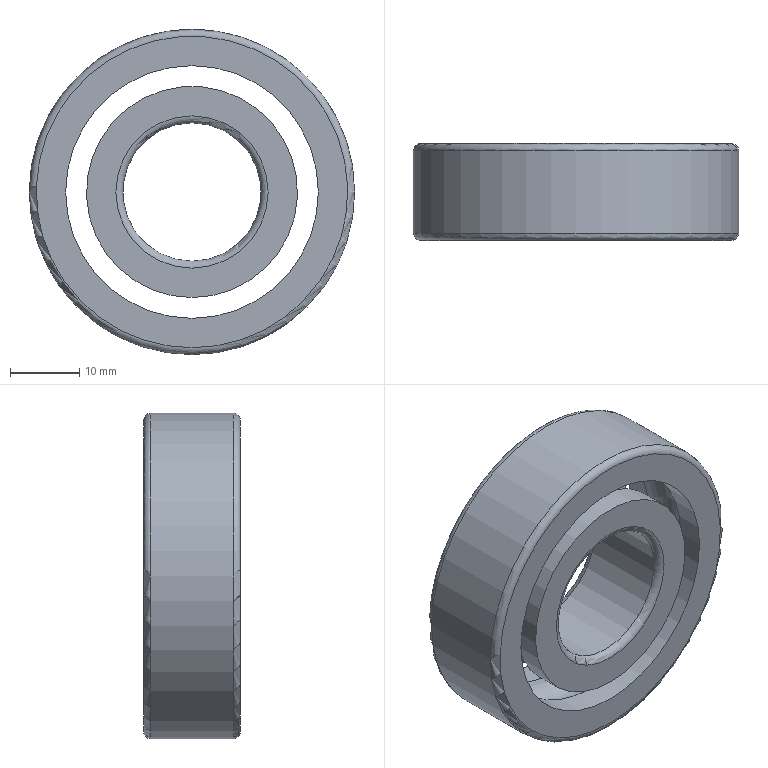Component | NX | GUNDONGZHOUCHENG9 | 2 solids | 16 faces | box 47 x 14 x 47 mm | volume 13471 mm3 | torus 6 | cylinder 6 | plane 4 | commonest cylinder face diameters 36.5 x2 30.5 x2 47 x1 20 x1
STEP:
#1=CARTESIAN_POINT('',(0.,0.,0.));
#2=DIRECTION('',(0.,0.,1.));
#3=DIRECTION('',(1.,0.,0.));
#4=AXIS2_PLACEMENT_3D('',#1,#2,#3);
#5=CARTESIAN_POINT('',(0.,0.,-22.5));
#6=VERTEX_POINT('',#5);
#7=CARTESIAN_POINT('',(0.,0.,0.));
#8=DIRECTION('',(0.,-1.,0.));
#9=DIRECTION('',(0.,0.,-1.));
#10=AXIS2_PLACEMENT_3D('',#7,#8,#9);
#11=CIRCLE('',#10,22.5);
#12=CARTESIAN_POINT('',(0.,1.,0.));
#13=DIRECTION('',(0.,-1.,0.));
#14=DIRECTION('',(0.,0.,-1.));
#15=AXIS2_PLACEMENT_3D('',#12,#13,#14);
#16=TOROIDAL_SURFACE('',#15,22.5,1.);
#17=CARTESIAN_POINT('',(0.,7.854));
#18=DIRECTION('',(1.,0.));
#19=VECTOR('',#18,1.);
#20=LINE('',#17,#19);
#21=(GEOMETRIC_REPRESENTATION_CONTEXT(2)PARAMETRIC_REPRESENTATION_CONTEXT()REPRESENTATION_CONTEXT('',''));
#22=DEFINITIONAL_REPRESENTATION('',(#20),#21);
#23=PCURVE('',#16,#22);
#24=CARTESIAN_POINT('',(22.5,0.,0.));
#25=DIRECTION('',(0.,1.,0.));
#26=DIRECTION('',(0.,0.,1.));
#27=AXIS2_PLACEMENT_3D('',#24,#25,#26);
#28=PLANE('',#27);
#29=CARTESIAN_POINT('',(-22.5,-22.5));
#30=CARTESIAN_POINT('',(-22.5,16.471));
#31=CARTESIAN_POINT('',(11.25,-3.014));
#32=CARTESIAN_POINT('',(45.,-22.5));
#33=CARTESIAN_POINT('',(11.25,-41.986));
#34=CARTESIAN_POINT('',(-22.5,-61.471));
#35=CARTESIAN_POINT('',(-22.5,-22.5));
#36=(BOUNDED_CURVE()B_SPLINE_CURVE(2,(#29,#30,#31,#32,#33,#34,#35),.UNSPECIFIED.,.T.,.F.)B_SPLINE_CURVE_WITH_KNOTS((1,2,2,2,2,1),(-2.094,0.,2.094,4.189,6.283,8.378),.UNSPECIFIED.)CURVE()GEOMETRIC_REPRESENTATION_ITEM()RATIONAL_B_SPLINE_CURVE((1.,0.5,1.,0.5,1.,0.5,1.))REPRESENTATION_ITEM(''));
#37=(GEOMETRIC_REPRESENTATION_CONTEXT(2)PARAMETRIC_REPRESENTATION_CONTEXT()REPRESENTATION_CONTEXT('',''));
#38=DEFINITIONAL_REPRESENTATION('',(#36),#37);
#39=PCURVE('',#28,#38);
#40=SURFACE_CURVE('',#11,(#23,#39),.PCURVE_S1.);
#41=EDGE_CURVE('',#6,#6,#40,.T.);
#42=ORIENTED_EDGE('',*,*,#41,.F.);
#43=CARTESIAN_POINT('',(0.,1.,-23.5));
#44=VERTEX_POINT('',#43);
#45=CARTESIAN_POINT('',(-0.,1.,-23.5));
#46=CARTESIAN_POINT('',(-0.,0.7327,-23.5));
#47=CARTESIAN_POINT('',(-0.,0.4723,-23.415));
#48=CARTESIAN_POINT('',(-0.,0.2481,-23.252));
#49=CARTESIAN_POINT('',(-0.,0.085,-23.028));
#50=CARTESIAN_POINT('',(-0.,0.,-22.767));
#51=CARTESIAN_POINT('',(-0.,0.,-22.5));
#52=(BOUNDED_CURVE()B_SPLINE_CURVE(6,(#45,#46,#47,#48,#49,#50,#51),.UNSPECIFIED.,.F.,.F.)B_SPLINE_CURVE_WITH_KNOTS((7,7),(0.,1.571),.PIECEWISE_BEZIER_KNOTS.)CURVE()GEOMETRIC_REPRESENTATION_ITEM()RATIONAL_B_SPLINE_CURVE((1.031,1.01,0.9979,0.994,0.9979,1.01,1.031))REPRESENTATION_ITEM(''));
#53=CARTESIAN_POINT('',(0.,6.283));
#54=DIRECTION('',(0.,1.));
#55=VECTOR('',#54,1.);
#56=LINE('',#53,#55);
#57=(GEOMETRIC_REPRESENTATION_CONTEXT(2)PARAMETRIC_REPRESENTATION_CONTEXT()REPRESENTATION_CONTEXT('',''));
#58=DEFINITIONAL_REPRESENTATION('',(#56),#57);
#59=PCURVE('',#16,#58);
#60=CARTESIAN_POINT('',(6.283,6.283));
#61=DIRECTION('',(0.,1.));
#62=VECTOR('',#61,1.);
#63=LINE('',#60,#62);
#64=(GEOMETRIC_REPRESENTATION_CONTEXT(2)PARAMETRIC_REPRESENTATION_CONTEXT()REPRESENTATION_CONTEXT('',''));
#65=DEFINITIONAL_REPRESENTATION('',(#63),#64);
#66=PCURVE('',#16,#65);
#67=SEAM_CURVE('',#52,(#59,#66),.PCURVE_S1.);
#68=EDGE_CURVE('',#44,#6,#67,.T.);
#69=ORIENTED_EDGE('',*,*,#68,.F.);
#70=CARTESIAN_POINT('',(0.,1.,0.));
#71=DIRECTION('',(0.,-1.,0.));
#72=DIRECTION('',(0.,0.,-1.));
#73=AXIS2_PLACEMENT_3D('',#70,#71,#72);
#74=CIRCLE('',#73,23.5);
#75=CARTESIAN_POINT('',(0.,6.283));
#76=DIRECTION('',(1.,0.));
#77=VECTOR('',#76,1.);
#78=LINE('',#75,#77);
#79=(GEOMETRIC_REPRESENTATION_CONTEXT(2)PARAMETRIC_REPRESENTATION_CONTEXT()REPRESENTATION_CONTEXT('',''));
#80=DEFINITIONAL_REPRESENTATION('',(#78),#79);
#81=PCURVE('',#16,#80);
#82=CARTESIAN_POINT('',(0.,0.,0.));
#83=DIRECTION('',(0.,-1.,0.));
#84=DIRECTION('',(0.,0.,-1.));
#85=AXIS2_PLACEMENT_3D('',#82,#83,#84);
#86=CYLINDRICAL_SURFACE('',#85,23.5);
#87=CARTESIAN_POINT('',(0.,-1.));
#88=DIRECTION('',(1.,0.));
#89=VECTOR('',#88,1.);
#90=LINE('',#87,#89);
#91=(GEOMETRIC_REPRESENTATION_CONTEXT(2)PARAMETRIC_REPRESENTATION_CONTEXT()REPRESENTATION_CONTEXT('',''));
#92=DEFINITIONAL_REPRESENTATION('',(#90),#91);
#93=PCURVE('',#86,#92);
#94=SURFACE_CURVE('',#74,(#81,#93),.PCURVE_S1.);
#95=EDGE_CURVE('',#44,#44,#94,.T.);
#96=ORIENTED_EDGE('',*,*,#95,.T.);
#97=ORIENTED_EDGE('',*,*,#68,.T.);
#98=EDGE_LOOP('',(#42,#69,#96,#97));
#99=FACE_BOUND('',#98,.T.);
#100=ADVANCED_FACE('',(#99),#16,.T.);
#101=CARTESIAN_POINT('',(0.,0.,-18.25));
#102=VERTEX_POINT('',#101);
#103=CARTESIAN_POINT('',(0.,0.,0.));
#104=DIRECTION('',(0.,-1.,0.));
#105=DIRECTION('',(0.,0.,-1.));
#106=AXIS2_PLACEMENT_3D('',#103,#104,#105);
#107=CIRCLE('',#106,18.25);
#108=CARTESIAN_POINT('',(-18.25,-22.5));
#109=CARTESIAN_POINT('',(-18.25,9.11));
#110=CARTESIAN_POINT('',(9.125,-6.695));
#111=CARTESIAN_POINT('',(36.5,-22.5));
#112=CARTESIAN_POINT('',(9.125,-38.305));
#113=CARTESIAN_POINT('',(-18.25,-54.11));
#114=CARTESIAN_POINT('',(-18.25,-22.5));
#115=(BOUNDED_CURVE()B_SPLINE_CURVE(2,(#108,#109,#110,#111,#112,#113,#114),.UNSPECIFIED.,.T.,.F.)B_SPLINE_CURVE_WITH_KNOTS((1,2,2,2,2,1),(-2.094,0.,2.094,4.189,6.283,8.378),.UNSPECIFIED.)CURVE()GEOMETRIC_REPRESENTATION_ITEM()RATIONAL_B_SPLINE_CURVE((1.,0.5,1.,0.5,1.,0.5,1.))REPRESENTATION_ITEM(''));
#116=(GEOMETRIC_REPRESENTATION_CONTEXT(2)PARAMETRIC_REPRESENTATION_CONTEXT()REPRESENTATION_CONTEXT('',''));
#117=DEFINITIONAL_REPRESENTATION('',(#115),#116);
#118=PCURVE('',#28,#117);
#119=CARTESIAN_POINT('',(0.,0.,0.));
#120=DIRECTION('',(0.,-1.,0.));
#121=DIRECTION('',(0.,0.,-1.));
#122=AXIS2_PLACEMENT_3D('',#119,#120,#121);
#123=CYLINDRICAL_SURFACE('',#122,18.25);
#124=CARTESIAN_POINT('',(0.,0.));
#125=DIRECTION('',(1.,0.));
#126=VECTOR('',#125,1.);
#127=LINE('',#124,#126);
#128=(GEOMETRIC_REPRESENTATION_CONTEXT(2)PARAMETRIC_REPRESENTATION_CONTEXT()REPRESENTATION_CONTEXT('',''));
#129=DEFINITIONAL_REPRESENTATION('',(#127),#128);
#130=PCURVE('',#123,#129);
#131=SURFACE_CURVE('',#107,(#118,#130),.PCURVE_S1.);
#132=EDGE_CURVE('',#102,#102,#131,.T.);
#133=ORIENTED_EDGE('',*,*,#132,.F.);
#134=EDGE_LOOP('',(#133));
#135=FACE_BOUND('',#134,.T.);
#136=ORIENTED_EDGE('',*,*,#41,.T.);
#137=EDGE_LOOP('',(#136));
#138=FACE_BOUND('',#137,.T.);
#139=ADVANCED_FACE('',(#135,#138),#28,.F.);
#140=CARTESIAN_POINT('',(0.,3.838,-18.25));
#141=VERTEX_POINT('',#140);
#142=CARTESIAN_POINT('',(0.,3.838,0.));
#143=DIRECTION('',(0.,-1.,0.));
#144=DIRECTION('',(0.,0.,-1.));
#145=AXIS2_PLACEMENT_3D('',#142,#143,#144);
#146=CIRCLE('',#145,18.25);
#147=CARTESIAN_POINT('',(0.,-3.838));
#148=DIRECTION('',(1.,0.));
#149=VECTOR('',#148,1.);
#150=LINE('',#147,#149);
#151=(GEOMETRIC_REPRESENTATION_CONTEXT(2)PARAMETRIC_REPRESENTATION_CONTEXT()REPRESENTATION_CONTEXT('',''));
#152=DEFINITIONAL_REPRESENTATION('',(#150),#151);
#153=PCURVE('',#123,#152);
#154=CARTESIAN_POINT('',(0.,7.,0.));
#155=DIRECTION('',(0.,-1.,0.));
#156=DIRECTION('',(0.,0.,-1.));
#157=AXIS2_PLACEMENT_3D('',#154,#155,#156);
#158=TOROIDAL_SURFACE('',#157,16.75,3.5);
#159=CARTESIAN_POINT('',(0.,7.411));
#160=DIRECTION('',(1.,0.));
#161=VECTOR('',#160,1.);
#162=LINE('',#159,#161);
#163=(GEOMETRIC_REPRESENTATION_CONTEXT(2)PARAMETRIC_REPRESENTATION_CONTEXT()REPRESENTATION_CONTEXT('',''));
#164=DEFINITIONAL_REPRESENTATION('',(#162),#163);
#165=PCURVE('',#158,#164);
#166=SURFACE_CURVE('',#146,(#153,#165),.PCURVE_S1.);
#167=EDGE_CURVE('',#141,#141,#166,.T.);
#168=ORIENTED_EDGE('',*,*,#167,.T.);
#169=CARTESIAN_POINT('',(0.,3.838,-18.25));
#170=CARTESIAN_POINT('',(0.,0.,-18.25));
#171=B_SPLINE_CURVE_WITH_KNOTS('',1,(#169,#170),.UNSPECIFIED.,.F.,.F.,(2,2),(-3.838,0.),.PIECEWISE_BEZIER_KNOTS.);
#172=CARTESIAN_POINT('',(6.283,0.));
#173=DIRECTION('',(0.,1.));
#174=VECTOR('',#173,1.);
#175=LINE('',#172,#174);
#176=(GEOMETRIC_REPRESENTATION_CONTEXT(2)PARAMETRIC_REPRESENTATION_CONTEXT()REPRESENTATION_CONTEXT('',''));
#177=DEFINITIONAL_REPRESENTATION('',(#175),#176);
#178=PCURVE('',#123,#177);
#179=CARTESIAN_POINT('',(0.,0.));
#180=DIRECTION('',(0.,1.));
#181=VECTOR('',#180,1.);
#182=LINE('',#179,#181);
#183=(GEOMETRIC_REPRESENTATION_CONTEXT(2)PARAMETRIC_REPRESENTATION_CONTEXT()REPRESENTATION_CONTEXT('',''));
#184=DEFINITIONAL_REPRESENTATION('',(#182),#183);
#185=PCURVE('',#123,#184);
#186=SEAM_CURVE('',#171,(#178,#185),.PCURVE_S1.);
#187=EDGE_CURVE('',#141,#102,#186,.T.);
#188=ORIENTED_EDGE('',*,*,#187,.T.);
#189=ORIENTED_EDGE('',*,*,#132,.F.);
#190=ORIENTED_EDGE('',*,*,#187,.F.);
#191=EDGE_LOOP('',(#168,#188,#189,#190));
#192=FACE_BOUND('',#191,.F.);
#193=ADVANCED_FACE('',(#192),#123,.F.);
#194=CARTESIAN_POINT('',(0.,10.162,-18.25));
#195=VERTEX_POINT('',#194);
#196=CARTESIAN_POINT('',(0.,10.162,0.));
#197=DIRECTION('',(0.,-1.,0.));
#198=DIRECTION('',(0.,0.,-1.));
#199=AXIS2_PLACEMENT_3D('',#196,#197,#198);
#200=CIRCLE('',#199,18.25);
#201=CARTESIAN_POINT('',(0.,5.155));
#202=DIRECTION('',(1.,0.));
#203=VECTOR('',#202,1.);
#204=LINE('',#201,#203);
#205=(GEOMETRIC_REPRESENTATION_CONTEXT(2)PARAMETRIC_REPRESENTATION_CONTEXT()REPRESENTATION_CONTEXT('',''));
#206=DEFINITIONAL_REPRESENTATION('',(#204),#205);
#207=PCURVE('',#158,#206);
#208=CARTESIAN_POINT('',(0.,0.,0.));
#209=DIRECTION('',(0.,-1.,0.));
#210=DIRECTION('',(0.,0.,-1.));
#211=AXIS2_PLACEMENT_3D('',#208,#209,#210);
#212=CYLINDRICAL_SURFACE('',#211,18.25);
#213=CARTESIAN_POINT('',(0.,-10.162));
#214=DIRECTION('',(1.,0.));
#215=VECTOR('',#214,1.);
#216=LINE('',#213,#215);
#217=(GEOMETRIC_REPRESENTATION_CONTEXT(2)PARAMETRIC_REPRESENTATION_CONTEXT()REPRESENTATION_CONTEXT('',''));
#218=DEFINITIONAL_REPRESENTATION('',(#216),#217);
#219=PCURVE('',#212,#218);
#220=SURFACE_CURVE('',#200,(#207,#219),.PCURVE_S1.);
#221=EDGE_CURVE('',#195,#195,#220,.T.);
#222=ORIENTED_EDGE('',*,*,#221,.T.);
#223=CARTESIAN_POINT('',(0.,10.162,-18.25));
#224=CARTESIAN_POINT('',(0.,9.679,-19.269));
#225=CARTESIAN_POINT('',(0.,8.812,-20.106));
#226=CARTESIAN_POINT('',(0.,7.645,-20.59));
#227=CARTESIAN_POINT('',(0.,6.355,-20.59));
#228=CARTESIAN_POINT('',(0.,5.188,-20.106));
#229=CARTESIAN_POINT('',(0.,4.321,-19.269));
#230=CARTESIAN_POINT('',(0.,3.838,-18.25));
#231=B_SPLINE_CURVE_WITH_KNOTS('',7,(#223,#224,#225,#226,#227,#228,#229,#230),.UNSPECIFIED.,.F.,.F.,(8,8),(5.155,7.411),.PIECEWISE_BEZIER_KNOTS.);
#232=CARTESIAN_POINT('',(6.283,0.));
#233=DIRECTION('',(0.,1.));
#234=VECTOR('',#233,1.);
#235=LINE('',#232,#234);
#236=(GEOMETRIC_REPRESENTATION_CONTEXT(2)PARAMETRIC_REPRESENTATION_CONTEXT()REPRESENTATION_CONTEXT('',''));
#237=DEFINITIONAL_REPRESENTATION('',(#235),#236);
#238=PCURVE('',#158,#237);
#239=CARTESIAN_POINT('',(0.,0.));
#240=DIRECTION('',(0.,1.));
#241=VECTOR('',#240,1.);
#242=LINE('',#239,#241);
#243=(GEOMETRIC_REPRESENTATION_CONTEXT(2)PARAMETRIC_REPRESENTATION_CONTEXT()REPRESENTATION_CONTEXT('',''));
#244=DEFINITIONAL_REPRESENTATION('',(#242),#243);
#245=PCURVE('',#158,#244);
#246=SEAM_CURVE('',#231,(#238,#245),.PCURVE_S1.);
#247=EDGE_CURVE('',#195,#141,#246,.T.);
#248=ORIENTED_EDGE('',*,*,#247,.T.);
#249=ORIENTED_EDGE('',*,*,#167,.F.);
#250=ORIENTED_EDGE('',*,*,#247,.F.);
#251=EDGE_LOOP('',(#222,#248,#249,#250));
#252=FACE_BOUND('',#251,.F.);
#253=ADVANCED_FACE('',(#252),#158,.F.);
#254=CARTESIAN_POINT('',(0.,14.,-18.25));
#255=VERTEX_POINT('',#254);
#256=CARTESIAN_POINT('',(0.,14.,0.));
#257=DIRECTION('',(0.,-1.,0.));
#258=DIRECTION('',(0.,0.,-1.));
#259=AXIS2_PLACEMENT_3D('',#256,#257,#258);
#260=CIRCLE('',#259,18.25);
#261=CARTESIAN_POINT('',(0.,-14.));
#262=DIRECTION('',(1.,0.));
#263=VECTOR('',#262,1.);
#264=LINE('',#261,#263);
#265=(GEOMETRIC_REPRESENTATION_CONTEXT(2)PARAMETRIC_REPRESENTATION_CONTEXT()REPRESENTATION_CONTEXT('',''));
#266=DEFINITIONAL_REPRESENTATION('',(#264),#265);
#267=PCURVE('',#212,#266);
#268=CARTESIAN_POINT('',(18.25,14.,0.));
#269=DIRECTION('',(0.,-1.,0.));
#270=DIRECTION('',(0.,0.,-1.));
#271=AXIS2_PLACEMENT_3D('',#268,#269,#270);
#272=PLANE('',#271);
#273=CARTESIAN_POINT('',(0.,-18.25));
#274=DIRECTION('',(1.,0.));
#275=AXIS2_PLACEMENT_2D('',#273,#274);
#276=CIRCLE('',#275,18.25);
#277=(GEOMETRIC_REPRESENTATION_CONTEXT(2)PARAMETRIC_REPRESENTATION_CONTEXT()REPRESENTATION_CONTEXT('',''));
#278=DEFINITIONAL_REPRESENTATION('',(#276),#277);
#279=PCURVE('',#272,#278);
#280=SURFACE_CURVE('',#260,(#267,#279),.PCURVE_S1.);
#281=EDGE_CURVE('',#255,#255,#280,.T.);
#282=ORIENTED_EDGE('',*,*,#281,.T.);
#283=CARTESIAN_POINT('',(0.,14.,-18.25));
#284=CARTESIAN_POINT('',(0.,10.162,-18.25));
#285=B_SPLINE_CURVE_WITH_KNOTS('',1,(#283,#284),.UNSPECIFIED.,.F.,.F.,(2,2),(-14.,-10.162),.PIECEWISE_BEZIER_KNOTS.);
#286=CARTESIAN_POINT('',(6.283,0.));
#287=DIRECTION('',(0.,1.));
#288=VECTOR('',#287,1.);
#289=LINE('',#286,#288);
#290=(GEOMETRIC_REPRESENTATION_CONTEXT(2)PARAMETRIC_REPRESENTATION_CONTEXT()REPRESENTATION_CONTEXT('',''));
#291=DEFINITIONAL_REPRESENTATION('',(#289),#290);
#292=PCURVE('',#212,#291);
#293=CARTESIAN_POINT('',(0.,0.));
#294=DIRECTION('',(0.,1.));
#295=VECTOR('',#294,1.);
#296=LINE('',#293,#295);
#297=(GEOMETRIC_REPRESENTATION_CONTEXT(2)PARAMETRIC_REPRESENTATION_CONTEXT()REPRESENTATION_CONTEXT('',''));
#298=DEFINITIONAL_REPRESENTATION('',(#296),#297);
#299=PCURVE('',#212,#298);
#300=SEAM_CURVE('',#285,(#292,#299),.PCURVE_S1.);
#301=EDGE_CURVE('',#255,#195,#300,.T.);
#302=ORIENTED_EDGE('',*,*,#301,.T.);
#303=ORIENTED_EDGE('',*,*,#221,.F.);
#304=ORIENTED_EDGE('',*,*,#301,.F.);
#305=EDGE_LOOP('',(#282,#302,#303,#304));
#306=FACE_BOUND('',#305,.F.);
#307=ADVANCED_FACE('',(#306),#212,.F.);
#308=CARTESIAN_POINT('',(0.,14.,-22.5));
#309=VERTEX_POINT('',#308);
#310=CARTESIAN_POINT('',(0.,14.,0.));
#311=DIRECTION('',(0.,-1.,0.));
#312=DIRECTION('',(0.,0.,-1.));
#313=AXIS2_PLACEMENT_3D('',#310,#311,#312);
#314=CIRCLE('',#313,22.5);
#315=CARTESIAN_POINT('',(0.,-18.25));
#316=DIRECTION('',(1.,0.));
#317=AXIS2_PLACEMENT_2D('',#315,#316);
#318=CIRCLE('',#317,22.5);
#319=(GEOMETRIC_REPRESENTATION_CONTEXT(2)PARAMETRIC_REPRESENTATION_CONTEXT()REPRESENTATION_CONTEXT('',''));
#320=DEFINITIONAL_REPRESENTATION('',(#318),#319);
#321=PCURVE('',#272,#320);
#322=CARTESIAN_POINT('',(0.,13.,0.));
#323=DIRECTION('',(0.,-1.,0.));
#324=DIRECTION('',(0.,0.,-1.));
#325=AXIS2_PLACEMENT_3D('',#322,#323,#324);
#326=TOROIDAL_SURFACE('',#325,22.5,1.);
#327=CARTESIAN_POINT('',(0.,4.712));
#328=DIRECTION('',(1.,0.));
#329=VECTOR('',#328,1.);
#330=LINE('',#327,#329);
#331=(GEOMETRIC_REPRESENTATION_CONTEXT(2)PARAMETRIC_REPRESENTATION_CONTEXT()REPRESENTATION_CONTEXT('',''));
#332=DEFINITIONAL_REPRESENTATION('',(#330),#331);
#333=PCURVE('',#326,#332);
#334=SURFACE_CURVE('',#314,(#321,#333),.PCURVE_S1.);
#335=EDGE_CURVE('',#309,#309,#334,.T.);
#336=ORIENTED_EDGE('',*,*,#335,.F.);
#337=EDGE_LOOP('',(#336));
#338=FACE_BOUND('',#337,.T.);
#339=ORIENTED_EDGE('',*,*,#281,.T.);
#340=EDGE_LOOP('',(#339));
#341=FACE_BOUND('',#340,.T.);
#342=ADVANCED_FACE('',(#338,#341),#272,.F.);
#343=CARTESIAN_POINT('',(0.,13.,-23.5));
#344=VERTEX_POINT('',#343);
#345=CARTESIAN_POINT('',(0.,13.,0.));
#346=DIRECTION('',(0.,-1.,0.));
#347=DIRECTION('',(0.,0.,-1.));
#348=AXIS2_PLACEMENT_3D('',#345,#346,#347);
#349=CIRCLE('',#348,23.5);
#350=CARTESIAN_POINT('',(0.,6.283));
#351=DIRECTION('',(1.,0.));
#352=VECTOR('',#351,1.);
#353=LINE('',#350,#352);
#354=(GEOMETRIC_REPRESENTATION_CONTEXT(2)PARAMETRIC_REPRESENTATION_CONTEXT()REPRESENTATION_CONTEXT('',''));
#355=DEFINITIONAL_REPRESENTATION('',(#353),#354);
#356=PCURVE('',#326,#355);
#357=CARTESIAN_POINT('',(0.,-13.));
#358=DIRECTION('',(1.,0.));
#359=VECTOR('',#358,1.);
#360=LINE('',#357,#359);
#361=(GEOMETRIC_REPRESENTATION_CONTEXT(2)PARAMETRIC_REPRESENTATION_CONTEXT()REPRESENTATION_CONTEXT('',''));
#362=DEFINITIONAL_REPRESENTATION('',(#360),#361);
#363=PCURVE('',#86,#362);
#364=SURFACE_CURVE('',#349,(#356,#363),.PCURVE_S1.);
#365=EDGE_CURVE('',#344,#344,#364,.T.);
#366=ORIENTED_EDGE('',*,*,#365,.F.);
#367=CARTESIAN_POINT('',(-0.,14.,-22.5));
#368=CARTESIAN_POINT('',(-0.,14.,-22.767));
#369=CARTESIAN_POINT('',(-0.,13.915,-23.028));
#370=CARTESIAN_POINT('',(-0.,13.752,-23.252));
#371=CARTESIAN_POINT('',(-0.,13.528,-23.415));
#372=CARTESIAN_POINT('',(-0.,13.267,-23.5));
#373=CARTESIAN_POINT('',(-0.,13.,-23.5));
#374=(BOUNDED_CURVE()B_SPLINE_CURVE(6,(#367,#368,#369,#370,#371,#372,#373),.UNSPECIFIED.,.F.,.F.)B_SPLINE_CURVE_WITH_KNOTS((7,7),(-1.571,0.),.PIECEWISE_BEZIER_KNOTS.)CURVE()GEOMETRIC_REPRESENTATION_ITEM()RATIONAL_B_SPLINE_CURVE((1.031,1.01,0.9979,0.994,0.9979,1.01,1.031))REPRESENTATION_ITEM(''));
#375=CARTESIAN_POINT('',(0.,6.283));
#376=DIRECTION('',(0.,1.));
#377=VECTOR('',#376,1.);
#378=LINE('',#375,#377);
#379=(GEOMETRIC_REPRESENTATION_CONTEXT(2)PARAMETRIC_REPRESENTATION_CONTEXT()REPRESENTATION_CONTEXT('',''));
#380=DEFINITIONAL_REPRESENTATION('',(#378),#379);
#381=PCURVE('',#326,#380);
#382=CARTESIAN_POINT('',(6.283,6.283));
#383=DIRECTION('',(0.,1.));
#384=VECTOR('',#383,1.);
#385=LINE('',#382,#384);
#386=(GEOMETRIC_REPRESENTATION_CONTEXT(2)PARAMETRIC_REPRESENTATION_CONTEXT()REPRESENTATION_CONTEXT('',''));
#387=DEFINITIONAL_REPRESENTATION('',(#385),#386);
#388=PCURVE('',#326,#387);
#389=SEAM_CURVE('',#374,(#381,#388),.PCURVE_S1.);
#390=EDGE_CURVE('',#309,#344,#389,.T.);
#391=ORIENTED_EDGE('',*,*,#390,.F.);
#392=ORIENTED_EDGE('',*,*,#335,.T.);
#393=ORIENTED_EDGE('',*,*,#390,.T.);
#394=EDGE_LOOP('',(#366,#391,#392,#393));
#395=FACE_BOUND('',#394,.T.);
#396=ADVANCED_FACE('',(#395),#326,.T.);
#397=ORIENTED_EDGE('',*,*,#95,.F.);
#398=CARTESIAN_POINT('',(-0.,13.,-23.5));
#399=CARTESIAN_POINT('',(-0.,1.,-23.5));
#400=B_SPLINE_CURVE_WITH_KNOTS('',1,(#398,#399),.UNSPECIFIED.,.F.,.F.,(2,2),(-13.,-1.),.PIECEWISE_BEZIER_KNOTS.);
#401=CARTESIAN_POINT('',(0.,0.));
#402=DIRECTION('',(0.,1.));
#403=VECTOR('',#402,1.);
#404=LINE('',#401,#403);
#405=(GEOMETRIC_REPRESENTATION_CONTEXT(2)PARAMETRIC_REPRESENTATION_CONTEXT()REPRESENTATION_CONTEXT('',''));
#406=DEFINITIONAL_REPRESENTATION('',(#404),#405);
#407=PCURVE('',#86,#406);
#408=CARTESIAN_POINT('',(6.283,0.));
#409=DIRECTION('',(0.,1.));
#410=VECTOR('',#409,1.);
#411=LINE('',#408,#410);
#412=(GEOMETRIC_REPRESENTATION_CONTEXT(2)PARAMETRIC_REPRESENTATION_CONTEXT()REPRESENTATION_CONTEXT('',''));
#413=DEFINITIONAL_REPRESENTATION('',(#411),#412);
#414=PCURVE('',#86,#413);
#415=SEAM_CURVE('',#400,(#407,#414),.PCURVE_S1.);
#416=EDGE_CURVE('',#344,#44,#415,.T.);
#417=ORIENTED_EDGE('',*,*,#416,.F.);
#418=ORIENTED_EDGE('',*,*,#365,.T.);
#419=ORIENTED_EDGE('',*,*,#416,.T.);
#420=EDGE_LOOP('',(#397,#417,#418,#419));
#421=FACE_BOUND('',#420,.T.);
#422=ADVANCED_FACE('',(#421),#86,.T.);
#423=CLOSED_SHELL('',(#100,#139,#193,#253,#307,#342,#396,#422));
#424=MANIFOLD_SOLID_BREP('',#423);
#425=(LENGTH_UNIT()NAMED_UNIT(*)SI_UNIT(.MILLI.,.METRE.));
#426=UNCERTAINTY_MEASURE_WITH_UNIT(LENGTH_MEASURE(0.00001),#425,'','');
#427=(NAMED_UNIT(*)PLANE_ANGLE_UNIT()SI_UNIT($,.RADIAN.));
#428=(NAMED_UNIT(*)SI_UNIT($,.STERADIAN.)SOLID_ANGLE_UNIT());
#429=(GEOMETRIC_REPRESENTATION_CONTEXT(3)GLOBAL_UNCERTAINTY_ASSIGNED_CONTEXT((#426))GLOBAL_UNIT_ASSIGNED_CONTEXT((#425,#427,#428))REPRESENTATION_CONTEXT('',''));
#430=ADVANCED_BREP_SHAPE_REPRESENTATION('',(#4,#424),#429);
#431=CARTESIAN_POINT('',(0.,0.,0.));
#432=DIRECTION('',(0.,0.,1.));
#433=DIRECTION('',(1.,0.,0.));
#434=AXIS2_PLACEMENT_3D('',#431,#432,#433);
#435=CARTESIAN_POINT('',(0.,0.,0.));
#436=DIRECTION('',(0.,0.,1.));
#437=DIRECTION('',(1.,0.,0.));
#438=AXIS2_PLACEMENT_3D('',#435,#436,#437);
#439=(LENGTH_UNIT()NAMED_UNIT(*)SI_UNIT(.MILLI.,.METRE.));
#440=UNCERTAINTY_MEASURE_WITH_UNIT(LENGTH_MEASURE(0.00001),#439,'','');
#441=(NAMED_UNIT(*)PLANE_ANGLE_UNIT()SI_UNIT($,.RADIAN.));
#442=(NAMED_UNIT(*)SI_UNIT($,.STERADIAN.)SOLID_ANGLE_UNIT());
#443=(GEOMETRIC_REPRESENTATION_CONTEXT(3)GLOBAL_UNCERTAINTY_ASSIGNED_CONTEXT((#440))GLOBAL_UNIT_ASSIGNED_CONTEXT((#439,#441,#442))REPRESENTATION_CONTEXT('',''));
#444=SHAPE_REPRESENTATION('',(#4,#434,#438),#443);
#445=ITEM_DEFINED_TRANSFORMATION('','',#4,#434);
#446=(REPRESENTATION_RELATIONSHIP('','',#430,#444)REPRESENTATION_RELATIONSHIP_WITH_TRANSFORMATION(#445)SHAPE_REPRESENTATION_RELATIONSHIP());
#447=CARTESIAN_POINT('',(0.,1.,-10.));
#448=VERTEX_POINT('',#447);
#449=CARTESIAN_POINT('',(0.,1.,0.));
#450=DIRECTION('',(0.,-1.,0.));
#451=DIRECTION('',(0.,0.,-1.));
#452=AXIS2_PLACEMENT_3D('',#449,#450,#451);
#453=CIRCLE('',#452,10.);
#454=CARTESIAN_POINT('',(0.,0.,0.));
#455=DIRECTION('',(0.,-1.,0.));
#456=DIRECTION('',(0.,0.,-1.));
#457=AXIS2_PLACEMENT_3D('',#454,#455,#456);
#458=CYLINDRICAL_SURFACE('',#457,10.);
#459=CARTESIAN_POINT('',(0.,-1.));
#460=DIRECTION('',(1.,0.));
#461=VECTOR('',#460,1.);
#462=LINE('',#459,#461);
#463=(GEOMETRIC_REPRESENTATION_CONTEXT(2)PARAMETRIC_REPRESENTATION_CONTEXT()REPRESENTATION_CONTEXT('',''));
#464=DEFINITIONAL_REPRESENTATION('',(#462),#463);
#465=PCURVE('',#458,#464);
#466=CARTESIAN_POINT('',(0.,1.,0.));
#467=DIRECTION('',(0.,-1.,0.));
#468=DIRECTION('',(0.,0.,-1.));
#469=AXIS2_PLACEMENT_3D('',#466,#467,#468);
#470=TOROIDAL_SURFACE('',#469,11.,1.);
#471=CARTESIAN_POINT('',(0.,9.425));
#472=DIRECTION('',(1.,0.));
#473=VECTOR('',#472,1.);
#474=LINE('',#471,#473);
#475=(GEOMETRIC_REPRESENTATION_CONTEXT(2)PARAMETRIC_REPRESENTATION_CONTEXT()REPRESENTATION_CONTEXT('',''));
#476=DEFINITIONAL_REPRESENTATION('',(#474),#475);
#477=PCURVE('',#470,#476);
#478=SURFACE_CURVE('',#453,(#465,#477),.PCURVE_S1.);
#479=EDGE_CURVE('',#448,#448,#478,.T.);
#480=ORIENTED_EDGE('',*,*,#479,.F.);
#481=CARTESIAN_POINT('',(0.,13.,-10.));
#482=VERTEX_POINT('',#481);
#483=CARTESIAN_POINT('',(-0.,13.,-10.));
#484=CARTESIAN_POINT('',(-0.,1.,-10.));
#485=B_SPLINE_CURVE_WITH_KNOTS('',1,(#483,#484),.UNSPECIFIED.,.F.,.F.,(2,2),(-13.,-1.),.PIECEWISE_BEZIER_KNOTS.);
#486=CARTESIAN_POINT('',(0.,0.));
#487=DIRECTION('',(0.,1.));
#488=VECTOR('',#487,1.);
#489=LINE('',#486,#488);
#490=(GEOMETRIC_REPRESENTATION_CONTEXT(2)PARAMETRIC_REPRESENTATION_CONTEXT()REPRESENTATION_CONTEXT('',''));
#491=DEFINITIONAL_REPRESENTATION('',(#489),#490);
#492=PCURVE('',#458,#491);
#493=CARTESIAN_POINT('',(6.283,0.));
#494=DIRECTION('',(0.,1.));
#495=VECTOR('',#494,1.);
#496=LINE('',#493,#495);
#497=(GEOMETRIC_REPRESENTATION_CONTEXT(2)PARAMETRIC_REPRESENTATION_CONTEXT()REPRESENTATION_CONTEXT('',''));
#498=DEFINITIONAL_REPRESENTATION('',(#496),#497);
#499=PCURVE('',#458,#498);
#500=SEAM_CURVE('',#485,(#492,#499),.PCURVE_S1.);
#501=EDGE_CURVE('',#482,#448,#500,.T.);
#502=ORIENTED_EDGE('',*,*,#501,.F.);
#503=CARTESIAN_POINT('',(0.,13.,0.));
#504=DIRECTION('',(0.,-1.,0.));
#505=DIRECTION('',(0.,0.,-1.));
#506=AXIS2_PLACEMENT_3D('',#503,#504,#505);
#507=CIRCLE('',#506,10.);
#508=CARTESIAN_POINT('',(0.,-13.));
#509=DIRECTION('',(1.,0.));
#510=VECTOR('',#509,1.);
#511=LINE('',#508,#510);
#512=(GEOMETRIC_REPRESENTATION_CONTEXT(2)PARAMETRIC_REPRESENTATION_CONTEXT()REPRESENTATION_CONTEXT('',''));
#513=DEFINITIONAL_REPRESENTATION('',(#511),#512);
#514=PCURVE('',#458,#513);
#515=CARTESIAN_POINT('',(0.,13.,0.));
#516=DIRECTION('',(0.,-1.,0.));
#517=DIRECTION('',(0.,0.,-1.));
#518=AXIS2_PLACEMENT_3D('',#515,#516,#517);
#519=TOROIDAL_SURFACE('',#518,11.,1.);
#520=CARTESIAN_POINT('',(0.,3.142));
#521=DIRECTION('',(1.,0.));
#522=VECTOR('',#521,1.);
#523=LINE('',#520,#522);
#524=(GEOMETRIC_REPRESENTATION_CONTEXT(2)PARAMETRIC_REPRESENTATION_CONTEXT()REPRESENTATION_CONTEXT('',''));
#525=DEFINITIONAL_REPRESENTATION('',(#523),#524);
#526=PCURVE('',#519,#525);
#527=SURFACE_CURVE('',#507,(#514,#526),.PCURVE_S1.);
#528=EDGE_CURVE('',#482,#482,#527,.T.);
#529=ORIENTED_EDGE('',*,*,#528,.T.);
#530=ORIENTED_EDGE('',*,*,#501,.T.);
#531=EDGE_LOOP('',(#480,#502,#529,#530));
#532=FACE_BOUND('',#531,.F.);
#533=ADVANCED_FACE('',(#532),#458,.F.);
#534=CARTESIAN_POINT('',(0.,0.,-11.));
#535=VERTEX_POINT('',#534);
#536=CARTESIAN_POINT('',(0.,0.,0.));
#537=DIRECTION('',(0.,-1.,0.));
#538=DIRECTION('',(0.,0.,-1.));
#539=AXIS2_PLACEMENT_3D('',#536,#537,#538);
#540=CIRCLE('',#539,11.);
#541=CARTESIAN_POINT('',(0.,7.854));
#542=DIRECTION('',(1.,0.));
#543=VECTOR('',#542,1.);
#544=LINE('',#541,#543);
#545=(GEOMETRIC_REPRESENTATION_CONTEXT(2)PARAMETRIC_REPRESENTATION_CONTEXT()REPRESENTATION_CONTEXT('',''));
#546=DEFINITIONAL_REPRESENTATION('',(#544),#545);
#547=PCURVE('',#470,#546);
#548=CARTESIAN_POINT('',(11.,0.,0.));
#549=DIRECTION('',(0.,-1.,0.));
#550=DIRECTION('',(0.,0.,-1.));
#551=AXIS2_PLACEMENT_3D('',#548,#549,#550);
#552=PLANE('',#551);
#553=CARTESIAN_POINT('',(0.,-11.));
#554=DIRECTION('',(1.,0.));
#555=AXIS2_PLACEMENT_2D('',#553,#554);
#556=CIRCLE('',#555,11.);
#557=(GEOMETRIC_REPRESENTATION_CONTEXT(2)PARAMETRIC_REPRESENTATION_CONTEXT()REPRESENTATION_CONTEXT('',''));
#558=DEFINITIONAL_REPRESENTATION('',(#556),#557);
#559=PCURVE('',#552,#558);
#560=SURFACE_CURVE('',#540,(#547,#559),.PCURVE_S1.);
#561=EDGE_CURVE('',#535,#535,#560,.T.);
#562=ORIENTED_EDGE('',*,*,#561,.T.);
#563=CARTESIAN_POINT('',(0.,0.,-11.));
#564=CARTESIAN_POINT('',(0.,0.,-10.733));
#565=CARTESIAN_POINT('',(0.,0.085,-10.472));
#566=CARTESIAN_POINT('',(0.,0.2481,-10.248));
#567=CARTESIAN_POINT('',(0.,0.4723,-10.085));
#568=CARTESIAN_POINT('',(0.,0.7327,-10.));
#569=CARTESIAN_POINT('',(0.,1.,-10.));
#570=(BOUNDED_CURVE()B_SPLINE_CURVE(6,(#563,#564,#565,#566,#567,#568,#569),.UNSPECIFIED.,.F.,.F.)B_SPLINE_CURVE_WITH_KNOTS((7,7),(1.571,3.142),.PIECEWISE_BEZIER_KNOTS.)CURVE()GEOMETRIC_REPRESENTATION_ITEM()RATIONAL_B_SPLINE_CURVE((1.031,1.01,0.9979,0.994,0.9979,1.01,1.031))REPRESENTATION_ITEM(''));
#571=CARTESIAN_POINT('',(6.283,6.283));
#572=DIRECTION('',(0.,1.));
#573=VECTOR('',#572,1.);
#574=LINE('',#571,#573);
#575=(GEOMETRIC_REPRESENTATION_CONTEXT(2)PARAMETRIC_REPRESENTATION_CONTEXT()REPRESENTATION_CONTEXT('',''));
#576=DEFINITIONAL_REPRESENTATION('',(#574),#575);
#577=PCURVE('',#470,#576);
#578=CARTESIAN_POINT('',(0.,6.283));
#579=DIRECTION('',(0.,1.));
#580=VECTOR('',#579,1.);
#581=LINE('',#578,#580);
#582=(GEOMETRIC_REPRESENTATION_CONTEXT(2)PARAMETRIC_REPRESENTATION_CONTEXT()REPRESENTATION_CONTEXT('',''));
#583=DEFINITIONAL_REPRESENTATION('',(#581),#582);
#584=PCURVE('',#470,#583);
#585=SEAM_CURVE('',#570,(#577,#584),.PCURVE_S1.);
#586=EDGE_CURVE('',#535,#448,#585,.T.);
#587=ORIENTED_EDGE('',*,*,#586,.T.);
#588=ORIENTED_EDGE('',*,*,#479,.F.);
#589=ORIENTED_EDGE('',*,*,#586,.F.);
#590=EDGE_LOOP('',(#562,#587,#588,#589));
#591=FACE_BOUND('',#590,.T.);
#592=ADVANCED_FACE('',(#591),#470,.T.);
#593=CARTESIAN_POINT('',(0.,0.,-15.25));
#594=VERTEX_POINT('',#593);
#595=CARTESIAN_POINT('',(0.,0.,0.));
#596=DIRECTION('',(0.,-1.,0.));
#597=DIRECTION('',(0.,0.,-1.));
#598=AXIS2_PLACEMENT_3D('',#595,#596,#597);
#599=CIRCLE('',#598,15.25);
#600=CARTESIAN_POINT('',(0.,-11.));
#601=DIRECTION('',(1.,0.));
#602=AXIS2_PLACEMENT_2D('',#600,#601);
#603=CIRCLE('',#602,15.25);
#604=(GEOMETRIC_REPRESENTATION_CONTEXT(2)PARAMETRIC_REPRESENTATION_CONTEXT()REPRESENTATION_CONTEXT('',''));
#605=DEFINITIONAL_REPRESENTATION('',(#603),#604);
#606=PCURVE('',#552,#605);
#607=CARTESIAN_POINT('',(0.,0.,0.));
#608=DIRECTION('',(0.,-1.,0.));
#609=DIRECTION('',(0.,0.,-1.));
#610=AXIS2_PLACEMENT_3D('',#607,#608,#609);
#611=CYLINDRICAL_SURFACE('',#610,15.25);
#612=CARTESIAN_POINT('',(0.,0.));
#613=DIRECTION('',(1.,0.));
#614=VECTOR('',#613,1.);
#615=LINE('',#612,#614);
#616=(GEOMETRIC_REPRESENTATION_CONTEXT(2)PARAMETRIC_REPRESENTATION_CONTEXT()REPRESENTATION_CONTEXT('',''));
#617=DEFINITIONAL_REPRESENTATION('',(#615),#616);
#618=PCURVE('',#611,#617);
#619=SURFACE_CURVE('',#599,(#606,#618),.PCURVE_S1.);
#620=EDGE_CURVE('',#594,#594,#619,.T.);
#621=ORIENTED_EDGE('',*,*,#620,.T.);
#622=EDGE_LOOP('',(#621));
#623=FACE_BOUND('',#622,.T.);
#624=ORIENTED_EDGE('',*,*,#561,.F.);
#625=EDGE_LOOP('',(#624));
#626=FACE_BOUND('',#625,.T.);
#627=ADVANCED_FACE('',(#623,#626),#552,.T.);
#628=CARTESIAN_POINT('',(0.,3.838,-15.25));
#629=VERTEX_POINT('',#628);
#630=CARTESIAN_POINT('',(0.,3.838,0.));
#631=DIRECTION('',(0.,-1.,0.));
#632=DIRECTION('',(0.,0.,-1.));
#633=AXIS2_PLACEMENT_3D('',#630,#631,#632);
#634=CIRCLE('',#633,15.25);
#635=CARTESIAN_POINT('',(0.,-3.838));
#636=DIRECTION('',(1.,0.));
#637=VECTOR('',#636,1.);
#638=LINE('',#635,#637);
#639=(GEOMETRIC_REPRESENTATION_CONTEXT(2)PARAMETRIC_REPRESENTATION_CONTEXT()REPRESENTATION_CONTEXT('',''));
#640=DEFINITIONAL_REPRESENTATION('',(#638),#639);
#641=PCURVE('',#611,#640);
#642=CARTESIAN_POINT('',(0.,7.,0.));
#643=DIRECTION('',(0.,-1.,0.));
#644=DIRECTION('',(0.,0.,-1.));
#645=AXIS2_PLACEMENT_3D('',#642,#643,#644);
#646=TOROIDAL_SURFACE('',#645,16.75,3.5);
#647=CARTESIAN_POINT('',(0.,2.014));
#648=DIRECTION('',(1.,0.));
#649=VECTOR('',#648,1.);
#650=LINE('',#647,#649);
#651=(GEOMETRIC_REPRESENTATION_CONTEXT(2)PARAMETRIC_REPRESENTATION_CONTEXT()REPRESENTATION_CONTEXT('',''));
#652=DEFINITIONAL_REPRESENTATION('',(#650),#651);
#653=PCURVE('',#646,#652);
#654=SURFACE_CURVE('',#634,(#641,#653),.PCURVE_S1.);
#655=EDGE_CURVE('',#629,#629,#654,.T.);
#656=ORIENTED_EDGE('',*,*,#655,.T.);
#657=CARTESIAN_POINT('',(0.,3.838,-15.25));
#658=CARTESIAN_POINT('',(0.,0.,-15.25));
#659=B_SPLINE_CURVE_WITH_KNOTS('',1,(#657,#658),.UNSPECIFIED.,.F.,.F.,(2,2),(-3.838,0.),.PIECEWISE_BEZIER_KNOTS.);
#660=CARTESIAN_POINT('',(6.283,0.));
#661=DIRECTION('',(0.,1.));
#662=VECTOR('',#661,1.);
#663=LINE('',#660,#662);
#664=(GEOMETRIC_REPRESENTATION_CONTEXT(2)PARAMETRIC_REPRESENTATION_CONTEXT()REPRESENTATION_CONTEXT('',''));
#665=DEFINITIONAL_REPRESENTATION('',(#663),#664);
#666=PCURVE('',#611,#665);
#667=CARTESIAN_POINT('',(0.,0.));
#668=DIRECTION('',(0.,1.));
#669=VECTOR('',#668,1.);
#670=LINE('',#667,#669);
#671=(GEOMETRIC_REPRESENTATION_CONTEXT(2)PARAMETRIC_REPRESENTATION_CONTEXT()REPRESENTATION_CONTEXT('',''));
#672=DEFINITIONAL_REPRESENTATION('',(#670),#671);
#673=PCURVE('',#611,#672);
#674=SEAM_CURVE('',#659,(#666,#673),.PCURVE_S1.);
#675=EDGE_CURVE('',#629,#594,#674,.T.);
#676=ORIENTED_EDGE('',*,*,#675,.T.);
#677=ORIENTED_EDGE('',*,*,#620,.F.);
#678=ORIENTED_EDGE('',*,*,#675,.F.);
#679=EDGE_LOOP('',(#656,#676,#677,#678));
#680=FACE_BOUND('',#679,.T.);
#681=ADVANCED_FACE('',(#680),#611,.T.);
#682=CARTESIAN_POINT('',(0.,10.162,-15.25));
#683=VERTEX_POINT('',#682);
#684=CARTESIAN_POINT('',(0.,10.162,0.));
#685=DIRECTION('',(0.,-1.,0.));
#686=DIRECTION('',(0.,0.,-1.));
#687=AXIS2_PLACEMENT_3D('',#684,#685,#686);
#688=CIRCLE('',#687,15.25);
#689=CARTESIAN_POINT('',(0.,4.269));
#690=DIRECTION('',(1.,0.));
#691=VECTOR('',#690,1.);
#692=LINE('',#689,#691);
#693=(GEOMETRIC_REPRESENTATION_CONTEXT(2)PARAMETRIC_REPRESENTATION_CONTEXT()REPRESENTATION_CONTEXT('',''));
#694=DEFINITIONAL_REPRESENTATION('',(#692),#693);
#695=PCURVE('',#646,#694);
#696=CARTESIAN_POINT('',(0.,0.,0.));
#697=DIRECTION('',(0.,-1.,0.));
#698=DIRECTION('',(0.,0.,-1.));
#699=AXIS2_PLACEMENT_3D('',#696,#697,#698);
#700=CYLINDRICAL_SURFACE('',#699,15.25);
#701=CARTESIAN_POINT('',(0.,-10.162));
#702=DIRECTION('',(1.,0.));
#703=VECTOR('',#702,1.);
#704=LINE('',#701,#703);
#705=(GEOMETRIC_REPRESENTATION_CONTEXT(2)PARAMETRIC_REPRESENTATION_CONTEXT()REPRESENTATION_CONTEXT('',''));
#706=DEFINITIONAL_REPRESENTATION('',(#704),#705);
#707=PCURVE('',#700,#706);
#708=SURFACE_CURVE('',#688,(#695,#707),.PCURVE_S1.);
#709=EDGE_CURVE('',#683,#683,#708,.T.);
#710=ORIENTED_EDGE('',*,*,#709,.F.);
#711=CARTESIAN_POINT('',(-0.,3.838,-15.25));
#712=CARTESIAN_POINT('',(-0.,4.427,-14.008));
#713=CARTESIAN_POINT('',(-0.,5.557,-13.108));
#714=CARTESIAN_POINT('',(-0.,7.,-12.779));
#715=CARTESIAN_POINT('',(-0.,8.443,-13.108));
#716=CARTESIAN_POINT('',(-0.,9.573,-14.008));
#717=CARTESIAN_POINT('',(-0.,10.162,-15.25));
#718=(BOUNDED_CURVE()B_SPLINE_CURVE(6,(#711,#712,#713,#714,#715,#716,#717),.UNSPECIFIED.,.F.,.F.)B_SPLINE_CURVE_WITH_KNOTS((7,7),(2.014,4.269),.PIECEWISE_BEZIER_KNOTS.)CURVE()GEOMETRIC_REPRESENTATION_ITEM()RATIONAL_B_SPLINE_CURVE((1.066,1.02,0.9958,0.9877,0.9958,1.02,1.066))REPRESENTATION_ITEM(''));
#719=CARTESIAN_POINT('',(0.,0.));
#720=DIRECTION('',(0.,1.));
#721=VECTOR('',#720,1.);
#722=LINE('',#719,#721);
#723=(GEOMETRIC_REPRESENTATION_CONTEXT(2)PARAMETRIC_REPRESENTATION_CONTEXT()REPRESENTATION_CONTEXT('',''));
#724=DEFINITIONAL_REPRESENTATION('',(#722),#723);
#725=PCURVE('',#646,#724);
#726=CARTESIAN_POINT('',(6.283,0.));
#727=DIRECTION('',(0.,1.));
#728=VECTOR('',#727,1.);
#729=LINE('',#726,#728);
#730=(GEOMETRIC_REPRESENTATION_CONTEXT(2)PARAMETRIC_REPRESENTATION_CONTEXT()REPRESENTATION_CONTEXT('',''));
#731=DEFINITIONAL_REPRESENTATION('',(#729),#730);
#732=PCURVE('',#646,#731);
#733=SEAM_CURVE('',#718,(#725,#732),.PCURVE_S1.);
#734=EDGE_CURVE('',#629,#683,#733,.T.);
#735=ORIENTED_EDGE('',*,*,#734,.F.);
#736=ORIENTED_EDGE('',*,*,#655,.T.);
#737=ORIENTED_EDGE('',*,*,#734,.T.);
#738=EDGE_LOOP('',(#710,#735,#736,#737));
#739=FACE_BOUND('',#738,.F.);
#740=ADVANCED_FACE('',(#739),#646,.F.);
#741=CARTESIAN_POINT('',(0.,14.,-15.25));
#742=VERTEX_POINT('',#741);
#743=CARTESIAN_POINT('',(0.,14.,0.));
#744=DIRECTION('',(0.,-1.,0.));
#745=DIRECTION('',(0.,0.,-1.));
#746=AXIS2_PLACEMENT_3D('',#743,#744,#745);
#747=CIRCLE('',#746,15.25);
#748=CARTESIAN_POINT('',(0.,-14.));
#749=DIRECTION('',(1.,0.));
#750=VECTOR('',#749,1.);
#751=LINE('',#748,#750);
#752=(GEOMETRIC_REPRESENTATION_CONTEXT(2)PARAMETRIC_REPRESENTATION_CONTEXT()REPRESENTATION_CONTEXT('',''));
#753=DEFINITIONAL_REPRESENTATION('',(#751),#752);
#754=PCURVE('',#700,#753);
#755=CARTESIAN_POINT('',(15.25,14.,0.));
#756=DIRECTION('',(0.,1.,0.));
#757=DIRECTION('',(0.,0.,1.));
#758=AXIS2_PLACEMENT_3D('',#755,#756,#757);
#759=PLANE('',#758);
#760=CARTESIAN_POINT('',(-15.25,-15.25));
#761=CARTESIAN_POINT('',(-15.25,11.164));
#762=CARTESIAN_POINT('',(7.625,-2.043));
#763=CARTESIAN_POINT('',(30.5,-15.25));
#764=CARTESIAN_POINT('',(7.625,-28.457));
#765=CARTESIAN_POINT('',(-15.25,-41.664));
#766=CARTESIAN_POINT('',(-15.25,-15.25));
#767=(BOUNDED_CURVE()B_SPLINE_CURVE(2,(#760,#761,#762,#763,#764,#765,#766),.UNSPECIFIED.,.T.,.F.)B_SPLINE_CURVE_WITH_KNOTS((1,2,2,2,2,1),(-2.094,0.,2.094,4.189,6.283,8.378),.UNSPECIFIED.)CURVE()GEOMETRIC_REPRESENTATION_ITEM()RATIONAL_B_SPLINE_CURVE((1.,0.5,1.,0.5,1.,0.5,1.))REPRESENTATION_ITEM(''));
#768=(GEOMETRIC_REPRESENTATION_CONTEXT(2)PARAMETRIC_REPRESENTATION_CONTEXT()REPRESENTATION_CONTEXT('',''));
#769=DEFINITIONAL_REPRESENTATION('',(#767),#768);
#770=PCURVE('',#759,#769);
#771=SURFACE_CURVE('',#747,(#754,#770),.PCURVE_S1.);
#772=EDGE_CURVE('',#742,#742,#771,.T.);
#773=ORIENTED_EDGE('',*,*,#772,.T.);
#774=CARTESIAN_POINT('',(0.,14.,-15.25));
#775=CARTESIAN_POINT('',(0.,10.162,-15.25));
#776=B_SPLINE_CURVE_WITH_KNOTS('',1,(#774,#775),.UNSPECIFIED.,.F.,.F.,(2,2),(-14.,-10.162),.PIECEWISE_BEZIER_KNOTS.);
#777=CARTESIAN_POINT('',(6.283,0.));
#778=DIRECTION('',(0.,1.));
#779=VECTOR('',#778,1.);
#780=LINE('',#777,#779);
#781=(GEOMETRIC_REPRESENTATION_CONTEXT(2)PARAMETRIC_REPRESENTATION_CONTEXT()REPRESENTATION_CONTEXT('',''));
#782=DEFINITIONAL_REPRESENTATION('',(#780),#781);
#783=PCURVE('',#700,#782);
#784=CARTESIAN_POINT('',(0.,0.));
#785=DIRECTION('',(0.,1.));
#786=VECTOR('',#785,1.);
#787=LINE('',#784,#786);
#788=(GEOMETRIC_REPRESENTATION_CONTEXT(2)PARAMETRIC_REPRESENTATION_CONTEXT()REPRESENTATION_CONTEXT('',''));
#789=DEFINITIONAL_REPRESENTATION('',(#787),#788);
#790=PCURVE('',#700,#789);
#791=SEAM_CURVE('',#776,(#783,#790),.PCURVE_S1.);
#792=EDGE_CURVE('',#742,#683,#791,.T.);
#793=ORIENTED_EDGE('',*,*,#792,.T.);
#794=ORIENTED_EDGE('',*,*,#709,.F.);
#795=ORIENTED_EDGE('',*,*,#792,.F.);
#796=EDGE_LOOP('',(#773,#793,#794,#795));
#797=FACE_BOUND('',#796,.T.);
#798=ADVANCED_FACE('',(#797),#700,.T.);
#799=CARTESIAN_POINT('',(0.,14.,-11.));
#800=VERTEX_POINT('',#799);
#801=CARTESIAN_POINT('',(0.,14.,0.));
#802=DIRECTION('',(0.,-1.,0.));
#803=DIRECTION('',(0.,0.,-1.));
#804=AXIS2_PLACEMENT_3D('',#801,#802,#803);
#805=CIRCLE('',#804,11.);
#806=CARTESIAN_POINT('',(-11.,-15.25));
#807=CARTESIAN_POINT('',(-11.,3.803));
#808=CARTESIAN_POINT('',(5.5,-5.724));
#809=CARTESIAN_POINT('',(22.,-15.25));
#810=CARTESIAN_POINT('',(5.5,-24.776));
#811=CARTESIAN_POINT('',(-11.,-34.303));
#812=CARTESIAN_POINT('',(-11.,-15.25));
#813=(BOUNDED_CURVE()B_SPLINE_CURVE(2,(#806,#807,#808,#809,#810,#811,#812),.UNSPECIFIED.,.T.,.F.)B_SPLINE_CURVE_WITH_KNOTS((1,2,2,2,2,1),(-2.094,0.,2.094,4.189,6.283,8.378),.UNSPECIFIED.)CURVE()GEOMETRIC_REPRESENTATION_ITEM()RATIONAL_B_SPLINE_CURVE((1.,0.5,1.,0.5,1.,0.5,1.))REPRESENTATION_ITEM(''));
#814=(GEOMETRIC_REPRESENTATION_CONTEXT(2)PARAMETRIC_REPRESENTATION_CONTEXT()REPRESENTATION_CONTEXT('',''));
#815=DEFINITIONAL_REPRESENTATION('',(#813),#814);
#816=PCURVE('',#759,#815);
#817=CARTESIAN_POINT('',(0.,4.712));
#818=DIRECTION('',(1.,0.));
#819=VECTOR('',#818,1.);
#820=LINE('',#817,#819);
#821=(GEOMETRIC_REPRESENTATION_CONTEXT(2)PARAMETRIC_REPRESENTATION_CONTEXT()REPRESENTATION_CONTEXT('',''));
#822=DEFINITIONAL_REPRESENTATION('',(#820),#821);
#823=PCURVE('',#519,#822);
#824=SURFACE_CURVE('',#805,(#816,#823),.PCURVE_S1.);
#825=EDGE_CURVE('',#800,#800,#824,.T.);
#826=ORIENTED_EDGE('',*,*,#825,.T.);
#827=EDGE_LOOP('',(#826));
#828=FACE_BOUND('',#827,.T.);
#829=ORIENTED_EDGE('',*,*,#772,.F.);
#830=EDGE_LOOP('',(#829));
#831=FACE_BOUND('',#830,.T.);
#832=ADVANCED_FACE('',(#828,#831),#759,.T.);
#833=ORIENTED_EDGE('',*,*,#528,.T.);
#834=CARTESIAN_POINT('',(0.,13.,-10.));
#835=CARTESIAN_POINT('',(0.,13.267,-10.));
#836=CARTESIAN_POINT('',(0.,13.528,-10.085));
#837=CARTESIAN_POINT('',(0.,13.752,-10.248));
#838=CARTESIAN_POINT('',(0.,13.915,-10.472));
#839=CARTESIAN_POINT('',(0.,14.,-10.733));
#840=CARTESIAN_POINT('',(0.,14.,-11.));
#841=(BOUNDED_CURVE()B_SPLINE_CURVE(6,(#834,#835,#836,#837,#838,#839,#840),.UNSPECIFIED.,.F.,.F.)B_SPLINE_CURVE_WITH_KNOTS((7,7),(3.142,4.712),.PIECEWISE_BEZIER_KNOTS.)CURVE()GEOMETRIC_REPRESENTATION_ITEM()RATIONAL_B_SPLINE_CURVE((1.031,1.01,0.9979,0.994,0.9979,1.01,1.031))REPRESENTATION_ITEM(''));
#842=CARTESIAN_POINT('',(6.283,0.));
#843=DIRECTION('',(0.,1.));
#844=VECTOR('',#843,1.);
#845=LINE('',#842,#844);
#846=(GEOMETRIC_REPRESENTATION_CONTEXT(2)PARAMETRIC_REPRESENTATION_CONTEXT()REPRESENTATION_CONTEXT('',''));
#847=DEFINITIONAL_REPRESENTATION('',(#845),#846);
#848=PCURVE('',#519,#847);
#849=CARTESIAN_POINT('',(0.,0.));
#850=DIRECTION('',(0.,1.));
#851=VECTOR('',#850,1.);
#852=LINE('',#849,#851);
#853=(GEOMETRIC_REPRESENTATION_CONTEXT(2)PARAMETRIC_REPRESENTATION_CONTEXT()REPRESENTATION_CONTEXT('',''));
#854=DEFINITIONAL_REPRESENTATION('',(#852),#853);
#855=PCURVE('',#519,#854);
#856=SEAM_CURVE('',#841,(#848,#855),.PCURVE_S1.);
#857=EDGE_CURVE('',#482,#800,#856,.T.);
#858=ORIENTED_EDGE('',*,*,#857,.T.);
#859=ORIENTED_EDGE('',*,*,#825,.F.);
#860=ORIENTED_EDGE('',*,*,#857,.F.);
#861=EDGE_LOOP('',(#833,#858,#859,#860));
#862=FACE_BOUND('',#861,.T.);
#863=ADVANCED_FACE('',(#862),#519,.T.);
#864=CLOSED_SHELL('',(#533,#592,#627,#681,#740,#798,#832,#863));
#865=MANIFOLD_SOLID_BREP('',#864);
#866=(LENGTH_UNIT()NAMED_UNIT(*)SI_UNIT(.MILLI.,.METRE.));
#867=UNCERTAINTY_MEASURE_WITH_UNIT(LENGTH_MEASURE(0.00001),#866,'','');
#868=(NAMED_UNIT(*)PLANE_ANGLE_UNIT()SI_UNIT($,.RADIAN.));
#869=(NAMED_UNIT(*)SI_UNIT($,.STERADIAN.)SOLID_ANGLE_UNIT());
#870=(GEOMETRIC_REPRESENTATION_CONTEXT(3)GLOBAL_UNCERTAINTY_ASSIGNED_CONTEXT((#867))GLOBAL_UNIT_ASSIGNED_CONTEXT((#866,#868,#869))REPRESENTATION_CONTEXT('',''));
#871=ADVANCED_BREP_SHAPE_REPRESENTATION('',(#4,#865),#870);
#872=ITEM_DEFINED_TRANSFORMATION('','',#4,#438);
#873=(REPRESENTATION_RELATIONSHIP('','',#871,#444)REPRESENTATION_RELATIONSHIP_WITH_TRANSFORMATION(#872)SHAPE_REPRESENTATION_RELATIONSHIP());